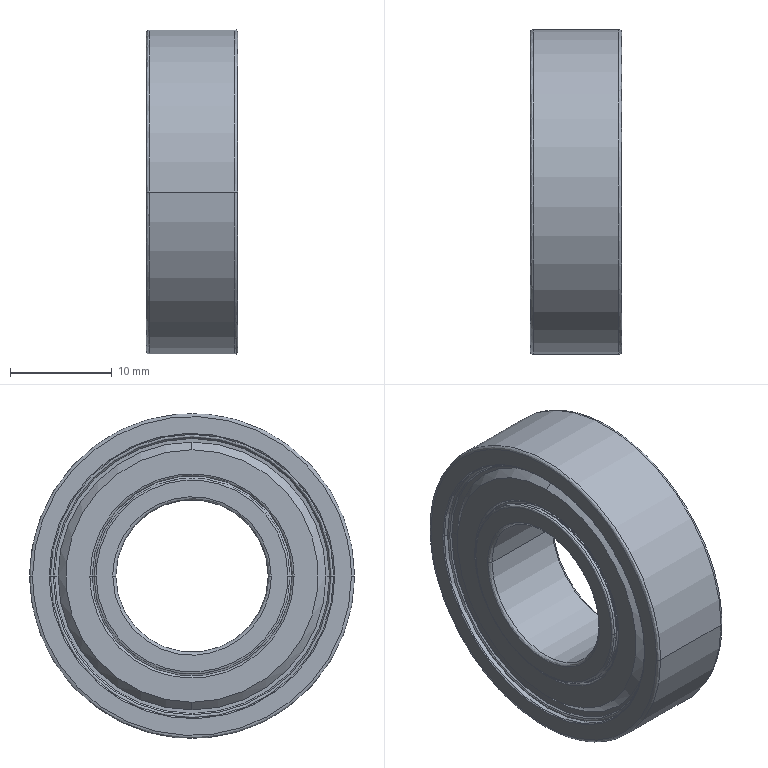Component | SolidWorks | Bearing6002Z-1 | 1 solid | 82 faces | volume 4557 mm3 | spline 32 | cylinder 22 | cone 20 | plane 8 | commonest cylinder face diameters 26.5 x4 20.5 x4 32 x2 27.9 x2 15 x2 19.3 x2 18.5 x2 19.7 x2 | material 45